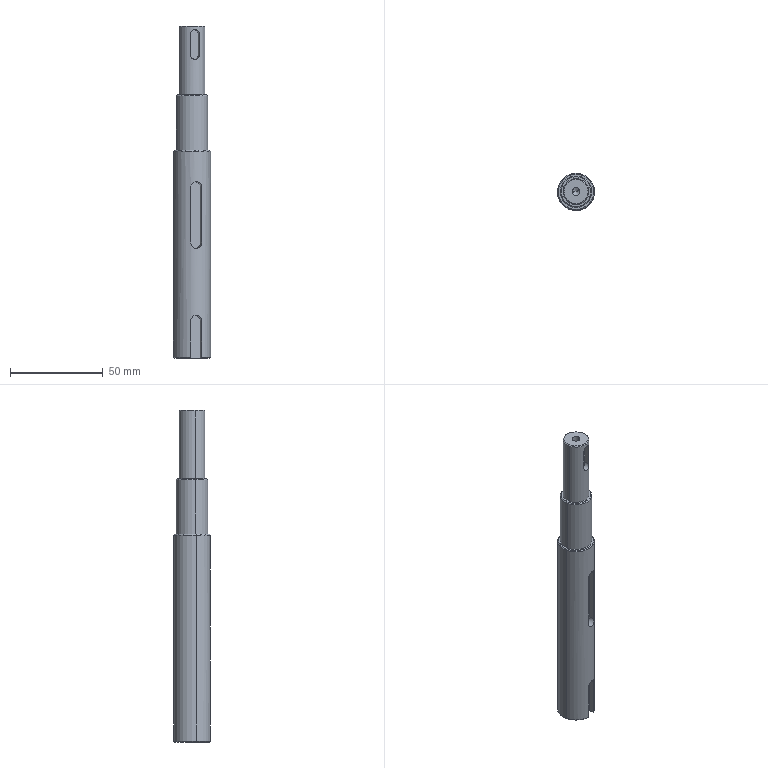Component | SolidWorks | Carrier1ZDG0406-A03-P83-X1-1 | 1 solid | 37 faces | box 20 x 20 x 179 mm | volume 46103 mm3 | cylinder 13 | plane 13 | cone 11 | commonest cylinder face diameters 6 x3 4.2 x2 20 x2 14 x2 17 x2 5 x2 | material Chrome Plated Rod
build123d program:
from build123d import *

# Parameters (mm, degrees)
CHAMFER1_SIZE         = 0.5
M5_TAPPED_HOLE2_D     = 4.2
M5_TAPPED_HOLE2_DEPTH = 14
M5_TAPPED_HOLE2_TIP   = 1.262
SKETCH10_W            = 336.857
SKETCH10_H            = 76.609
CUT_EXTRUDE2_DEPTH    = 50.5
CHAMFER2_SIZE         = 0.5
CUT_EXTRUDE3_DEPTH    = 3.5
KEYSEAT_B5_L15_DEPTH  = 3


with BuildPart() as part:
    # Sketch1_2 → Revolve1 (revolve)
    with BuildSketch(Plane.XY, mode=Mode.PRIVATE) as revolve1_sk:
        Polygon((-134, 10), (226, 10), (226, 8.5), (256, 8.5), (256, 7), (293, 7), (293, 0), (-143, 0), (-143, 8.5), (-134, 8.5), align=None)
    revolve(revolve1_sk.sketch.rotate(Axis((-324.043, 0, 0), (1, 0, 0)), 90), axis=Axis((-324.043, 0, 0), (1, 0, 0)))

    # Chamfer1
    chamfer1_edges = [part.edges().sort_by_distance(p)[0] for p in [
        (256, 0, -8.5),
        (226, 0, -10),
        (-134, 0, -10),
        (-143, 0, -8.5),
        (293, 0, -7),
    ]]
    chamfer(chamfer1_edges, length=CHAMFER1_SIZE)

    # M5 Tapped Hole2
    with Locations(Plane(origin=(293, 1.08, 1.659), x_dir=(0, 0, -1), z_dir=(1, 0, 0))):
        with Locations((1.659, -1.08)):
            Hole(M5_TAPPED_HOLE2_D / 2, depth=M5_TAPPED_HOLE2_DEPTH)
            with Locations((0, 0, -(M5_TAPPED_HOLE2_DEPTH + M5_TAPPED_HOLE2_TIP / 2))):  # 118° drill point
                Cone(0, M5_TAPPED_HOLE2_D / 2, M5_TAPPED_HOLE2_TIP, mode=Mode.SUBTRACT)

    # Sketch10 → Cut-Extrude2 (cut, symmetric)
    with BuildSketch(Plane(origin=(0, 0, 0), x_dir=(1, 0, 0), z_dir=(0, 1, 0))):
        with Locations((-54.429, 3.639)):
            Rectangle(SKETCH10_W, SKETCH10_H)
    extrude(amount=CUT_EXTRUDE2_DEPTH, both=True, mode=Mode.SUBTRACT)

    # Chamfer2
    chamfer2_edges = [part.edges().sort_by_distance(p)[0] for p in [
        (114, 0, -10),
    ]]
    chamfer(chamfer2_edges, length=CHAMFER2_SIZE)

    # Sketch11 → Cut-Extrude3 (cut)
    with BuildSketch(Plane(origin=(0, 10, 0), x_dir=(1, 0, 0), z_dir=(0, 1, 0))):
        with BuildLine():
            Line((176, 3), (206, 3))
            ThreePointArc((206, 3), (209, 0), (206, -3))
            Line((206, -3), (176, -3))
            ThreePointArc((176, -3), (173, 0), (176, 3))
        make_face()
        with BuildLine():
            Line((114, 3), (134, 3))
            ThreePointArc((134, 3), (137, 0), (134, -3))
            Line((134, -3), (114, -3))
            ThreePointArc((114, -3), (111, 0), (114, 3))
        make_face()
    extrude(amount=-CUT_EXTRUDE3_DEPTH, mode=Mode.SUBTRACT)

    # Sketch1 → Keyseat-B5-L15 (cut)
    with BuildSketch(Plane(origin=(0, 7, 0), x_dir=(1, 0, 0), z_dir=(0, 1, 0))):
        with BuildLine():
            Line((277.5, 2.5), (288.5, 2.5))
            ThreePointArc((288.5, 2.5), (291, 0), (288.5, -2.5))
            Line((288.5, -2.5), (277.5, -2.5))
            ThreePointArc((277.5, -2.5), (275, 0), (277.5, 2.5))
        make_face()
    extrude(amount=-KEYSEAT_B5_L15_DEPTH, mode=Mode.SUBTRACT)


solid = part.part

# Placed as in the assembly
solid = solid.moved(Location((-22.5, 0, -241), (-90, 76.275, -90)))